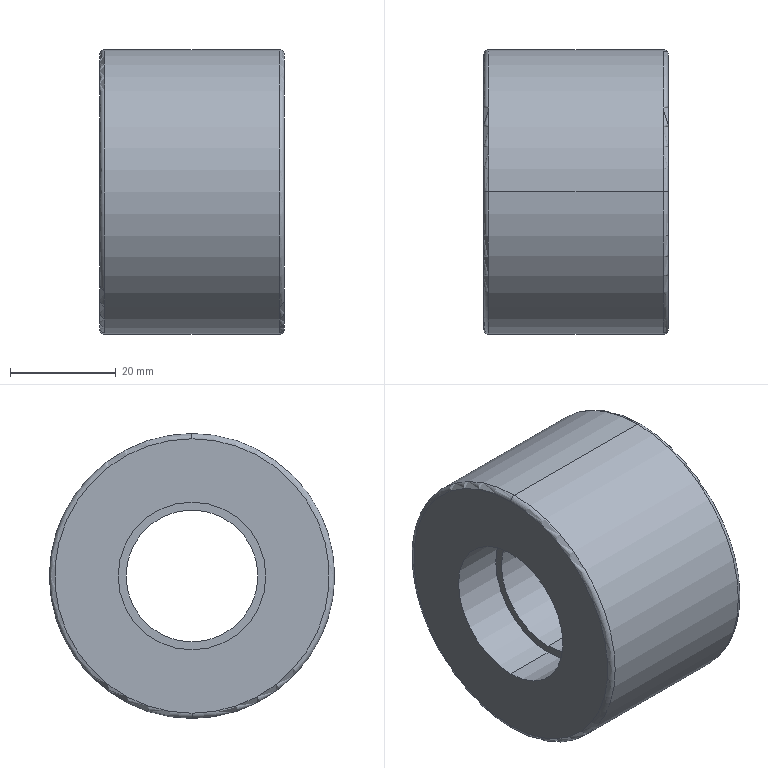Component | SolidWorks | CHEN123-AA-09-1 | 1 solid | 16 faces | box 35 x 54 x 54 mm | volume 60407 mm3 | cylinder 8 | torus 4 | plane 4 | commonest cylinder face diameters 28 x4 54 x2 25 x2
build123d program:
from build123d import *

# Parameters (mm, degrees)
SKETCH1_R           = 27
BOSS_EXTRUDE1_DEPTH = 17.5
SKETCH2_R           = 12.5
CUT_EXTRUDE1_DEPTH  = 52.798
SKETCH3_R           = 14
CUT_EXTRUDE2_DEPTH  = 10
CUT_EXTRUDE3_START  = -10
SKETCH4_R           = 14
CUT_EXTRUDE3_DEPTH  = 10
FILLET1_R           = 1


with BuildPart() as part:
    # Sketch1 → Boss-Extrude1 (new, symmetric)
    with BuildSketch(Plane.XY):
        Circle(SKETCH1_R)
    extrude(amount=BOSS_EXTRUDE1_DEPTH, both=True)

    # Sketch2 → Cut-Extrude1 (cut, through all)
    with BuildSketch(Plane.XY.offset(17.5)):
        Circle(SKETCH2_R)
    extrude(amount=-CUT_EXTRUDE1_DEPTH, mode=Mode.SUBTRACT)

    # Sketch3 → Cut-Extrude2 (cut)
    with BuildSketch(Plane.XY.offset(17.5)):
        Circle(SKETCH3_R)
    extrude(amount=-CUT_EXTRUDE2_DEPTH, mode=Mode.SUBTRACT)

    # Sketch4 → Cut-Extrude3 (cut)
    with BuildSketch(Plane(origin=(0, 0, -17.5), x_dir=(-1, 0, 0), z_dir=(0, 0, -1)).offset(CUT_EXTRUDE3_START)):
        with Locations(Location((0, 0, 0), (0, 0, 180))):
            Circle(SKETCH4_R)
    extrude(amount=CUT_EXTRUDE3_DEPTH, mode=Mode.SUBTRACT)

    # Fillet1
    fillet1_edges = [part.edges().sort_by_distance(p)[0] for p in [
        (-27, 0, -17.5),
        (-27, 0, 17.5),
    ]]
    fillet(fillet1_edges, radius=FILLET1_R)


solid = part.part

# Placed as in the assembly
solid = solid.moved(Location((-0.0005, 4.001, 34), (0, 90, 0)))
STEP:
#1=COLOUR_RGB('',0.7922,0.8196,0.9333);
#2=FILL_AREA_STYLE_COLOUR('',#1);
#3=FILL_AREA_STYLE('',(#2));
#4=SURFACE_STYLE_FILL_AREA(#3);
#5=SURFACE_SIDE_STYLE('',(#4));
#6=SURFACE_STYLE_USAGE(.BOTH.,#5);
#7=PRESENTATION_STYLE_ASSIGNMENT((#6));
#8=CARTESIAN_POINT('',(0.6496,0.1575,2.402));
#9=VERTEX_POINT('',#8);
#10=CARTESIAN_POINT('',(0.6496,0.1575,0.2756));
#11=VERTEX_POINT('',#10);
#12=CARTESIAN_POINT('',(0.6496,0.1575,1.339));
#13=DIRECTION('',(-1.,0.,0.));
#14=DIRECTION('',(0.,0.,-1.));
#15=AXIS2_PLACEMENT_3D('',#12,#13,#14);
#16=CIRCLE('',#15,1.063);
#17=EDGE_CURVE('',#9,#11,#16,.T.);
#18=ORIENTED_EDGE('',*,*,#17,.F.);
#19=CARTESIAN_POINT('',(0.689,0.1575,2.362));
#20=VERTEX_POINT('',#19);
#21=CARTESIAN_POINT('',(0.6496,0.1575,2.362));
#22=DIRECTION('',(0.,1.,-0.));
#23=DIRECTION('',(0.,0.,1.));
#24=AXIS2_PLACEMENT_3D('',#21,#22,#23);
#25=CIRCLE('',#24,0.03937);
#26=EDGE_CURVE('',#9,#20,#25,.T.);
#27=ORIENTED_EDGE('',*,*,#26,.T.);
#28=CARTESIAN_POINT('',(0.689,0.1575,0.315));
#29=VERTEX_POINT('',#28);
#30=CARTESIAN_POINT('',(0.689,0.1575,1.339));
#31=DIRECTION('',(1.,0.,0.));
#32=DIRECTION('',(0.,0.,-1.));
#33=AXIS2_PLACEMENT_3D('',#30,#31,#32);
#34=CIRCLE('',#33,1.024);
#35=EDGE_CURVE('',#29,#20,#34,.T.);
#36=ORIENTED_EDGE('',*,*,#35,.F.);
#37=CARTESIAN_POINT('',(0.6496,0.1575,0.315));
#38=DIRECTION('',(0.,-1.,0.));
#39=DIRECTION('',(0.,0.,-1.));
#40=AXIS2_PLACEMENT_3D('',#37,#38,#39);
#41=CIRCLE('',#40,0.03937);
#42=EDGE_CURVE('',#11,#29,#41,.T.);
#43=ORIENTED_EDGE('',*,*,#42,.F.);
#44=EDGE_LOOP('',(#18,#27,#36,#43));
#45=FACE_OUTER_BOUND('',#44,.T.);
#46=CARTESIAN_POINT('',(0.6496,0.1575,1.339));
#47=DIRECTION('',(1.,0.,0.));
#48=DIRECTION('',(0.,0.,-1.));
#49=AXIS2_PLACEMENT_3D('',#46,#47,#48);
#50=TOROIDAL_SURFACE('',#49,1.024,0.03937);
#51=ADVANCED_FACE('',(#45),#50,.T.);
#52=CARTESIAN_POINT('',(-0.689,0.1575,2.362));
#53=VERTEX_POINT('',#52);
#54=CARTESIAN_POINT('',(-0.689,0.1575,0.315));
#55=VERTEX_POINT('',#54);
#56=CARTESIAN_POINT('',(-0.689,0.1575,1.339));
#57=DIRECTION('',(-1.,0.,0.));
#58=DIRECTION('',(0.,0.,-1.));
#59=AXIS2_PLACEMENT_3D('',#56,#57,#58);
#60=CIRCLE('',#59,1.024);
#61=EDGE_CURVE('',#53,#55,#60,.T.);
#62=ORIENTED_EDGE('',*,*,#61,.F.);
#63=CARTESIAN_POINT('',(-0.6496,0.1575,2.402));
#64=VERTEX_POINT('',#63);
#65=CARTESIAN_POINT('',(-0.6496,0.1575,2.362));
#66=DIRECTION('',(0.,1.,-0.));
#67=DIRECTION('',(0.,0.,1.));
#68=AXIS2_PLACEMENT_3D('',#65,#66,#67);
#69=CIRCLE('',#68,0.03937);
#70=EDGE_CURVE('',#53,#64,#69,.T.);
#71=ORIENTED_EDGE('',*,*,#70,.T.);
#72=CARTESIAN_POINT('',(-0.6496,0.1575,0.2756));
#73=VERTEX_POINT('',#72);
#74=CARTESIAN_POINT('',(-0.6496,0.1575,1.339));
#75=DIRECTION('',(1.,0.,0.));
#76=DIRECTION('',(0.,0.,-1.));
#77=AXIS2_PLACEMENT_3D('',#74,#75,#76);
#78=CIRCLE('',#77,1.063);
#79=EDGE_CURVE('',#73,#64,#78,.T.);
#80=ORIENTED_EDGE('',*,*,#79,.F.);
#81=CARTESIAN_POINT('',(-0.6496,0.1575,0.315));
#82=DIRECTION('',(0.,-1.,0.));
#83=DIRECTION('',(0.,0.,-1.));
#84=AXIS2_PLACEMENT_3D('',#81,#82,#83);
#85=CIRCLE('',#84,0.03937);
#86=EDGE_CURVE('',#55,#73,#85,.T.);
#87=ORIENTED_EDGE('',*,*,#86,.F.);
#88=EDGE_LOOP('',(#62,#71,#80,#87));
#89=FACE_OUTER_BOUND('',#88,.T.);
#90=CARTESIAN_POINT('',(-0.6496,0.1575,1.339));
#91=DIRECTION('',(1.,0.,0.));
#92=DIRECTION('',(0.,0.,-1.));
#93=AXIS2_PLACEMENT_3D('',#90,#91,#92);
#94=TOROIDAL_SURFACE('',#93,1.024,0.03937);
#95=ADVANCED_FACE('',(#89),#94,.T.);
#96=CARTESIAN_POINT('',(-0.2953,0.1575,0.7874));
#97=VERTEX_POINT('',#96);
#98=CARTESIAN_POINT('',(-0.2953,0.1575,1.89));
#99=VERTEX_POINT('',#98);
#100=CARTESIAN_POINT('',(-0.2953,0.1575,1.339));
#101=DIRECTION('',(-1.,0.,0.));
#102=DIRECTION('',(0.,0.,1.));
#103=AXIS2_PLACEMENT_3D('',#100,#101,#102);
#104=CIRCLE('',#103,0.5512);
#105=EDGE_CURVE('',#97,#99,#104,.T.);
#106=ORIENTED_EDGE('',*,*,#105,.F.);
#107=CARTESIAN_POINT('',(-0.689,0.1575,0.7874));
#108=VERTEX_POINT('',#107);
#109=CARTESIAN_POINT('',(-0.2953,0.1575,0.7874));
#110=DIRECTION('',(-1.,0.,0.));
#111=VECTOR('',#110,39.37);
#112=LINE('',#109,#111);
#113=EDGE_CURVE('',#97,#108,#112,.T.);
#114=ORIENTED_EDGE('',*,*,#113,.T.);
#115=CARTESIAN_POINT('',(-0.689,0.1575,1.89));
#116=VERTEX_POINT('',#115);
#117=CARTESIAN_POINT('',(-0.689,0.1575,1.339));
#118=DIRECTION('',(-1.,0.,0.));
#119=DIRECTION('',(0.,0.,1.));
#120=AXIS2_PLACEMENT_3D('',#117,#118,#119);
#121=CIRCLE('',#120,0.5512);
#122=EDGE_CURVE('',#108,#116,#121,.T.);
#123=ORIENTED_EDGE('',*,*,#122,.T.);
#124=CARTESIAN_POINT('',(-0.2953,0.1575,1.89));
#125=DIRECTION('',(-1.,0.,0.));
#126=VECTOR('',#125,39.37);
#127=LINE('',#124,#126);
#128=EDGE_CURVE('',#99,#116,#127,.T.);
#129=ORIENTED_EDGE('',*,*,#128,.F.);
#130=EDGE_LOOP('',(#106,#114,#123,#129));
#131=FACE_OUTER_BOUND('',#130,.T.);
#132=CARTESIAN_POINT('',(-0.2953,0.1575,1.339));
#133=DIRECTION('',(-1.,0.,0.));
#134=DIRECTION('',(0.,0.,1.));
#135=AXIS2_PLACEMENT_3D('',#132,#133,#134);
#136=CYLINDRICAL_SURFACE('',#135,0.5512);
#137=ADVANCED_FACE('',(#131),#136,.F.);
#138=CARTESIAN_POINT('',(0.2953,0.1575,1.89));
#139=VERTEX_POINT('',#138);
#140=CARTESIAN_POINT('',(0.2953,0.1575,0.7874));
#141=VERTEX_POINT('',#140);
#142=CARTESIAN_POINT('',(0.2953,0.1575,1.339));
#143=DIRECTION('',(1.,0.,0.));
#144=DIRECTION('',(0.,0.,-1.));
#145=AXIS2_PLACEMENT_3D('',#142,#143,#144);
#146=CIRCLE('',#145,0.5512);
#147=EDGE_CURVE('',#139,#141,#146,.T.);
#148=ORIENTED_EDGE('',*,*,#147,.F.);
#149=CARTESIAN_POINT('',(0.689,0.1575,1.89));
#150=VERTEX_POINT('',#149);
#151=CARTESIAN_POINT('',(0.2953,0.1575,1.89));
#152=DIRECTION('',(1.,0.,0.));
#153=VECTOR('',#152,39.37);
#154=LINE('',#151,#153);
#155=EDGE_CURVE('',#139,#150,#154,.T.);
#156=ORIENTED_EDGE('',*,*,#155,.T.);
#157=CARTESIAN_POINT('',(0.689,0.1575,0.7874));
#158=VERTEX_POINT('',#157);
#159=CARTESIAN_POINT('',(0.689,0.1575,1.339));
#160=DIRECTION('',(1.,0.,0.));
#161=DIRECTION('',(0.,0.,-1.));
#162=AXIS2_PLACEMENT_3D('',#159,#160,#161);
#163=CIRCLE('',#162,0.5512);
#164=EDGE_CURVE('',#150,#158,#163,.T.);
#165=ORIENTED_EDGE('',*,*,#164,.T.);
#166=CARTESIAN_POINT('',(0.2953,0.1575,0.7874));
#167=DIRECTION('',(1.,0.,0.));
#168=VECTOR('',#167,39.37);
#169=LINE('',#166,#168);
#170=EDGE_CURVE('',#141,#158,#169,.T.);
#171=ORIENTED_EDGE('',*,*,#170,.F.);
#172=EDGE_LOOP('',(#148,#156,#165,#171));
#173=FACE_OUTER_BOUND('',#172,.T.);
#174=CARTESIAN_POINT('',(0.2953,0.1575,1.339));
#175=DIRECTION('',(1.,0.,0.));
#176=DIRECTION('',(0.,0.,-1.));
#177=AXIS2_PLACEMENT_3D('',#174,#175,#176);
#178=CYLINDRICAL_SURFACE('',#177,0.5512);
#179=ADVANCED_FACE('',(#173),#178,.F.);
#180=ORIENTED_EDGE('',*,*,#17,.T.);
#181=CARTESIAN_POINT('',(0.689,0.1575,0.2756));
#182=DIRECTION('',(-1.,0.,0.));
#183=VECTOR('',#182,39.37);
#184=LINE('',#181,#183);
#185=EDGE_CURVE('',#11,#73,#184,.T.);
#186=ORIENTED_EDGE('',*,*,#185,.T.);
#187=ORIENTED_EDGE('',*,*,#79,.T.);
#188=CARTESIAN_POINT('',(0.689,0.1575,2.402));
#189=DIRECTION('',(-1.,0.,0.));
#190=VECTOR('',#189,39.37);
#191=LINE('',#188,#190);
#192=EDGE_CURVE('',#9,#64,#191,.T.);
#193=ORIENTED_EDGE('',*,*,#192,.F.);
#194=EDGE_LOOP('',(#180,#186,#187,#193));
#195=FACE_OUTER_BOUND('',#194,.T.);
#196=CARTESIAN_POINT('',(0.689,0.1575,1.339));
#197=DIRECTION('',(-1.,0.,0.));
#198=DIRECTION('',(0.,0.,1.));
#199=AXIS2_PLACEMENT_3D('',#196,#197,#198);
#200=CYLINDRICAL_SURFACE('',#199,1.063);
#201=ADVANCED_FACE('',(#195),#200,.T.);
#202=CARTESIAN_POINT('',(-0.2953,0.1575,1.831));
#203=VERTEX_POINT('',#202);
#204=CARTESIAN_POINT('',(-0.2953,0.1575,0.8465));
#205=VERTEX_POINT('',#204);
#206=CARTESIAN_POINT('',(-0.2953,0.1575,1.339));
#207=DIRECTION('',(1.,0.,0.));
#208=DIRECTION('',(0.,0.,1.));
#209=AXIS2_PLACEMENT_3D('',#206,#207,#208);
#210=CIRCLE('',#209,0.4921);
#211=EDGE_CURVE('',#203,#205,#210,.T.);
#212=ORIENTED_EDGE('',*,*,#211,.F.);
#213=CARTESIAN_POINT('',(0.2953,0.1575,1.831));
#214=VERTEX_POINT('',#213);
#215=CARTESIAN_POINT('',(-0.689,0.1575,1.831));
#216=DIRECTION('',(1.,0.,0.));
#217=VECTOR('',#216,39.37);
#218=LINE('',#215,#217);
#219=EDGE_CURVE('',#203,#214,#218,.T.);
#220=ORIENTED_EDGE('',*,*,#219,.T.);
#221=CARTESIAN_POINT('',(0.2953,0.1575,0.8465));
#222=VERTEX_POINT('',#221);
#223=CARTESIAN_POINT('',(0.2953,0.1575,1.339));
#224=DIRECTION('',(-1.,0.,0.));
#225=DIRECTION('',(0.,0.,-1.));
#226=AXIS2_PLACEMENT_3D('',#223,#224,#225);
#227=CIRCLE('',#226,0.4921);
#228=EDGE_CURVE('',#222,#214,#227,.T.);
#229=ORIENTED_EDGE('',*,*,#228,.F.);
#230=CARTESIAN_POINT('',(-0.689,0.1575,0.8465));
#231=DIRECTION('',(1.,0.,0.));
#232=VECTOR('',#231,39.37);
#233=LINE('',#230,#232);
#234=EDGE_CURVE('',#205,#222,#233,.T.);
#235=ORIENTED_EDGE('',*,*,#234,.F.);
#236=EDGE_LOOP('',(#212,#220,#229,#235));
#237=FACE_OUTER_BOUND('',#236,.T.);
#238=CARTESIAN_POINT('',(-0.689,0.1575,1.339));
#239=DIRECTION('',(1.,0.,0.));
#240=DIRECTION('',(0.,0.,-1.));
#241=AXIS2_PLACEMENT_3D('',#238,#239,#240);
#242=CYLINDRICAL_SURFACE('',#241,0.4921);
#243=ADVANCED_FACE('',(#237),#242,.F.);
#244=ORIENTED_EDGE('',*,*,#219,.F.);
#245=CARTESIAN_POINT('',(-0.2953,0.1575,1.339));
#246=DIRECTION('',(1.,0.,0.));
#247=DIRECTION('',(0.,0.,1.));
#248=AXIS2_PLACEMENT_3D('',#245,#246,#247);
#249=CIRCLE('',#248,0.4921);
#250=EDGE_CURVE('',#205,#203,#249,.T.);
#251=ORIENTED_EDGE('',*,*,#250,.F.);
#252=ORIENTED_EDGE('',*,*,#234,.T.);
#253=CARTESIAN_POINT('',(0.2953,0.1575,1.339));
#254=DIRECTION('',(-1.,0.,0.));
#255=DIRECTION('',(0.,0.,-1.));
#256=AXIS2_PLACEMENT_3D('',#253,#254,#255);
#257=CIRCLE('',#256,0.4921);
#258=EDGE_CURVE('',#214,#222,#257,.T.);
#259=ORIENTED_EDGE('',*,*,#258,.F.);
#260=EDGE_LOOP('',(#244,#251,#252,#259));
#261=FACE_OUTER_BOUND('',#260,.T.);
#262=CARTESIAN_POINT('',(-0.689,0.1575,1.339));
#263=DIRECTION('',(1.,0.,0.));
#264=DIRECTION('',(0.,0.,-1.));
#265=AXIS2_PLACEMENT_3D('',#262,#263,#264);
#266=CYLINDRICAL_SURFACE('',#265,0.4921);
#267=ADVANCED_FACE('',(#261),#266,.F.);
#268=ORIENTED_EDGE('',*,*,#185,.F.);
#269=CARTESIAN_POINT('',(0.6496,0.1575,1.339));
#270=DIRECTION('',(-1.,0.,0.));
#271=DIRECTION('',(0.,0.,-1.));
#272=AXIS2_PLACEMENT_3D('',#269,#270,#271);
#273=CIRCLE('',#272,1.063);
#274=EDGE_CURVE('',#11,#9,#273,.T.);
#275=ORIENTED_EDGE('',*,*,#274,.T.);
#276=ORIENTED_EDGE('',*,*,#192,.T.);
#277=CARTESIAN_POINT('',(-0.6496,0.1575,1.339));
#278=DIRECTION('',(1.,0.,0.));
#279=DIRECTION('',(0.,0.,-1.));
#280=AXIS2_PLACEMENT_3D('',#277,#278,#279);
#281=CIRCLE('',#280,1.063);
#282=EDGE_CURVE('',#64,#73,#281,.T.);
#283=ORIENTED_EDGE('',*,*,#282,.T.);
#284=EDGE_LOOP('',(#268,#275,#276,#283));
#285=FACE_OUTER_BOUND('',#284,.T.);
#286=CARTESIAN_POINT('',(0.689,0.1575,1.339));
#287=DIRECTION('',(-1.,0.,0.));
#288=DIRECTION('',(0.,0.,1.));
#289=AXIS2_PLACEMENT_3D('',#286,#287,#288);
#290=CYLINDRICAL_SURFACE('',#289,1.063);
#291=ADVANCED_FACE('',(#285),#290,.T.);
#292=ORIENTED_EDGE('',*,*,#35,.T.);
#293=CARTESIAN_POINT('',(0.689,0.1575,1.339));
#294=DIRECTION('',(1.,0.,0.));
#295=DIRECTION('',(0.,0.,-1.));
#296=AXIS2_PLACEMENT_3D('',#293,#294,#295);
#297=CIRCLE('',#296,1.024);
#298=EDGE_CURVE('',#20,#29,#297,.T.);
#299=ORIENTED_EDGE('',*,*,#298,.T.);
#300=EDGE_LOOP('',(#292,#299));
#301=FACE_OUTER_BOUND('',#300,.T.);
#302=CARTESIAN_POINT('',(0.689,0.1575,1.339));
#303=DIRECTION('',(1.,0.,0.));
#304=DIRECTION('',(0.,0.,-1.));
#305=AXIS2_PLACEMENT_3D('',#302,#303,#304);
#306=CIRCLE('',#305,0.5512);
#307=EDGE_CURVE('',#158,#150,#306,.T.);
#308=ORIENTED_EDGE('',*,*,#307,.F.);
#309=ORIENTED_EDGE('',*,*,#164,.F.);
#310=EDGE_LOOP('',(#308,#309));
#311=FACE_BOUND('',#310,.T.);
#312=CARTESIAN_POINT('',(0.689,0.1575,1.339));
#313=DIRECTION('',(1.,0.,0.));
#314=DIRECTION('',(0.,0.,-1.));
#315=AXIS2_PLACEMENT_3D('',#312,#313,#314);
#316=PLANE('',#315);
#317=ADVANCED_FACE('',(#301,#311),#316,.T.);
#318=CARTESIAN_POINT('',(-0.689,0.1575,1.339));
#319=DIRECTION('',(-1.,0.,0.));
#320=DIRECTION('',(0.,0.,-1.));
#321=AXIS2_PLACEMENT_3D('',#318,#319,#320);
#322=CIRCLE('',#321,1.024);
#323=EDGE_CURVE('',#55,#53,#322,.T.);
#324=ORIENTED_EDGE('',*,*,#323,.T.);
#325=ORIENTED_EDGE('',*,*,#61,.T.);
#326=EDGE_LOOP('',(#324,#325));
#327=FACE_OUTER_BOUND('',#326,.T.);
#328=CARTESIAN_POINT('',(-0.689,0.1575,1.339));
#329=DIRECTION('',(-1.,0.,0.));
#330=DIRECTION('',(0.,0.,1.));
#331=AXIS2_PLACEMENT_3D('',#328,#329,#330);
#332=CIRCLE('',#331,0.5512);
#333=EDGE_CURVE('',#116,#108,#332,.T.);
#334=ORIENTED_EDGE('',*,*,#333,.F.);
#335=ORIENTED_EDGE('',*,*,#122,.F.);
#336=EDGE_LOOP('',(#334,#335));
#337=FACE_BOUND('',#336,.T.);
#338=CARTESIAN_POINT('',(-0.689,0.1575,1.339));
#339=DIRECTION('',(1.,0.,0.));
#340=DIRECTION('',(0.,0.,-1.));
#341=AXIS2_PLACEMENT_3D('',#338,#339,#340);
#342=PLANE('',#341);
#343=ADVANCED_FACE('',(#327,#337),#342,.F.);
#344=CARTESIAN_POINT('',(0.2953,0.1575,1.339));
#345=DIRECTION('',(1.,0.,0.));
#346=DIRECTION('',(0.,0.,-1.));
#347=AXIS2_PLACEMENT_3D('',#344,#345,#346);
#348=CIRCLE('',#347,0.5512);
#349=EDGE_CURVE('',#141,#139,#348,.T.);
#350=ORIENTED_EDGE('',*,*,#349,.T.);
#351=ORIENTED_EDGE('',*,*,#147,.T.);
#352=EDGE_LOOP('',(#350,#351));
#353=FACE_OUTER_BOUND('',#352,.T.);
#354=ORIENTED_EDGE('',*,*,#228,.T.);
#355=ORIENTED_EDGE('',*,*,#258,.T.);
#356=EDGE_LOOP('',(#354,#355));
#357=FACE_BOUND('',#356,.T.);
#358=CARTESIAN_POINT('',(0.2953,0.1575,1.339));
#359=DIRECTION('',(1.,0.,0.));
#360=DIRECTION('',(0.,0.,-1.));
#361=AXIS2_PLACEMENT_3D('',#358,#359,#360);
#362=PLANE('',#361);
#363=ADVANCED_FACE('',(#353,#357),#362,.T.);
#364=ORIENTED_EDGE('',*,*,#155,.F.);
#365=ORIENTED_EDGE('',*,*,#349,.F.);
#366=ORIENTED_EDGE('',*,*,#170,.T.);
#367=ORIENTED_EDGE('',*,*,#307,.T.);
#368=EDGE_LOOP('',(#364,#365,#366,#367));
#369=FACE_OUTER_BOUND('',#368,.T.);
#370=CARTESIAN_POINT('',(0.2953,0.1575,1.339));
#371=DIRECTION('',(1.,0.,0.));
#372=DIRECTION('',(0.,0.,-1.));
#373=AXIS2_PLACEMENT_3D('',#370,#371,#372);
#374=CYLINDRICAL_SURFACE('',#373,0.5512);
#375=ADVANCED_FACE('',(#369),#374,.F.);
#376=CARTESIAN_POINT('',(-0.2953,0.1575,1.339));
#377=DIRECTION('',(-1.,0.,0.));
#378=DIRECTION('',(0.,0.,1.));
#379=AXIS2_PLACEMENT_3D('',#376,#377,#378);
#380=CIRCLE('',#379,0.5512);
#381=EDGE_CURVE('',#99,#97,#380,.T.);
#382=ORIENTED_EDGE('',*,*,#381,.T.);
#383=ORIENTED_EDGE('',*,*,#105,.T.);
#384=EDGE_LOOP('',(#382,#383));
#385=FACE_OUTER_BOUND('',#384,.T.);
#386=ORIENTED_EDGE('',*,*,#250,.T.);
#387=ORIENTED_EDGE('',*,*,#211,.T.);
#388=EDGE_LOOP('',(#386,#387));
#389=FACE_BOUND('',#388,.T.);
#390=CARTESIAN_POINT('',(-0.2953,0.1575,1.339));
#391=DIRECTION('',(-1.,0.,0.));
#392=DIRECTION('',(0.,0.,1.));
#393=AXIS2_PLACEMENT_3D('',#390,#391,#392);
#394=PLANE('',#393);
#395=ADVANCED_FACE('',(#385,#389),#394,.T.);
#396=ORIENTED_EDGE('',*,*,#113,.F.);
#397=ORIENTED_EDGE('',*,*,#381,.F.);
#398=ORIENTED_EDGE('',*,*,#128,.T.);
#399=ORIENTED_EDGE('',*,*,#333,.T.);
#400=EDGE_LOOP('',(#396,#397,#398,#399));
#401=FACE_OUTER_BOUND('',#400,.T.);
#402=CARTESIAN_POINT('',(-0.2953,0.1575,1.339));
#403=DIRECTION('',(-1.,0.,0.));
#404=DIRECTION('',(0.,0.,1.));
#405=AXIS2_PLACEMENT_3D('',#402,#403,#404);
#406=CYLINDRICAL_SURFACE('',#405,0.5512);
#407=ADVANCED_FACE('',(#401),#406,.F.);
#408=ORIENTED_EDGE('',*,*,#70,.F.);
#409=ORIENTED_EDGE('',*,*,#323,.F.);
#410=ORIENTED_EDGE('',*,*,#86,.T.);
#411=ORIENTED_EDGE('',*,*,#282,.F.);
#412=EDGE_LOOP('',(#408,#409,#410,#411));
#413=FACE_OUTER_BOUND('',#412,.T.);
#414=CARTESIAN_POINT('',(-0.6496,0.1575,1.339));
#415=DIRECTION('',(1.,0.,0.));
#416=DIRECTION('',(0.,0.,-1.));
#417=AXIS2_PLACEMENT_3D('',#414,#415,#416);
#418=TOROIDAL_SURFACE('',#417,1.024,0.03937);
#419=ADVANCED_FACE('',(#413),#418,.T.);
#420=ORIENTED_EDGE('',*,*,#26,.F.);
#421=ORIENTED_EDGE('',*,*,#274,.F.);
#422=ORIENTED_EDGE('',*,*,#42,.T.);
#423=ORIENTED_EDGE('',*,*,#298,.F.);
#424=EDGE_LOOP('',(#420,#421,#422,#423));
#425=FACE_OUTER_BOUND('',#424,.T.);
#426=CARTESIAN_POINT('',(0.6496,0.1575,1.339));
#427=DIRECTION('',(1.,0.,0.));
#428=DIRECTION('',(0.,0.,-1.));
#429=AXIS2_PLACEMENT_3D('',#426,#427,#428);
#430=TOROIDAL_SURFACE('',#429,1.024,0.03937);
#431=ADVANCED_FACE('',(#425),#430,.T.);
#432=CLOSED_SHELL('',(#51,#95,#137,#179,#201,#243,#267,#291,#317,#343,#363,#375,#395,#407,#419,#431));
#433=MANIFOLD_SOLID_BREP('',#432);
#434=STYLED_ITEM('',(#7),#433);
#435=(LENGTH_UNIT()NAMED_UNIT(*)SI_UNIT($,.METRE.));
#436=LENGTH_MEASURE_WITH_UNIT(LENGTH_MEASURE(0.0254),#435);
#437=DIMENSIONAL_EXPONENTS(1.,0.,0.,0.,0.,0.,0.);
#438=(CONVERSION_BASED_UNIT('',#436)LENGTH_UNIT()NAMED_UNIT(#437));
#439=UNCERTAINTY_MEASURE_WITH_UNIT(LENGTH_MEASURE(0.00001),#438,'','');
#440=(NAMED_UNIT(*)PLANE_ANGLE_UNIT()SI_UNIT($,.RADIAN.));
#441=(NAMED_UNIT(*)SI_UNIT($,.STERADIAN.)SOLID_ANGLE_UNIT());
#442=(GEOMETRIC_REPRESENTATION_CONTEXT(3)GLOBAL_UNCERTAINTY_ASSIGNED_CONTEXT((#439))GLOBAL_UNIT_ASSIGNED_CONTEXT((#438,#440,#441))REPRESENTATION_CONTEXT('',''));
#443=MECHANICAL_DESIGN_GEOMETRIC_PRESENTATION_REPRESENTATION('',(#434),#442);
#444=CARTESIAN_POINT('',(0.,0.,0.));
#445=DIRECTION('',(0.,0.,1.));
#446=DIRECTION('',(1.,0.,0.));
#447=AXIS2_PLACEMENT_3D('',#444,#445,#446);
#448=(LENGTH_UNIT()NAMED_UNIT(*)SI_UNIT($,.METRE.));
#449=LENGTH_MEASURE_WITH_UNIT(LENGTH_MEASURE(0.0254),#448);
#450=DIMENSIONAL_EXPONENTS(1.,0.,0.,0.,0.,0.,0.);
#451=(CONVERSION_BASED_UNIT('',#449)LENGTH_UNIT()NAMED_UNIT(#450));
#452=UNCERTAINTY_MEASURE_WITH_UNIT(LENGTH_MEASURE(0.00001),#451,'','');
#453=(NAMED_UNIT(*)PLANE_ANGLE_UNIT()SI_UNIT($,.RADIAN.));
#454=(NAMED_UNIT(*)SI_UNIT($,.STERADIAN.)SOLID_ANGLE_UNIT());
#455=(GEOMETRIC_REPRESENTATION_CONTEXT(3)GLOBAL_UNCERTAINTY_ASSIGNED_CONTEXT((#452))GLOBAL_UNIT_ASSIGNED_CONTEXT((#451,#453,#454))REPRESENTATION_CONTEXT('',''));
#456=ADVANCED_BREP_SHAPE_REPRESENTATION('',(#433,#447),#455);
#457=PRESENTATION_LAYER_ASSIGNMENT('','',(#434));